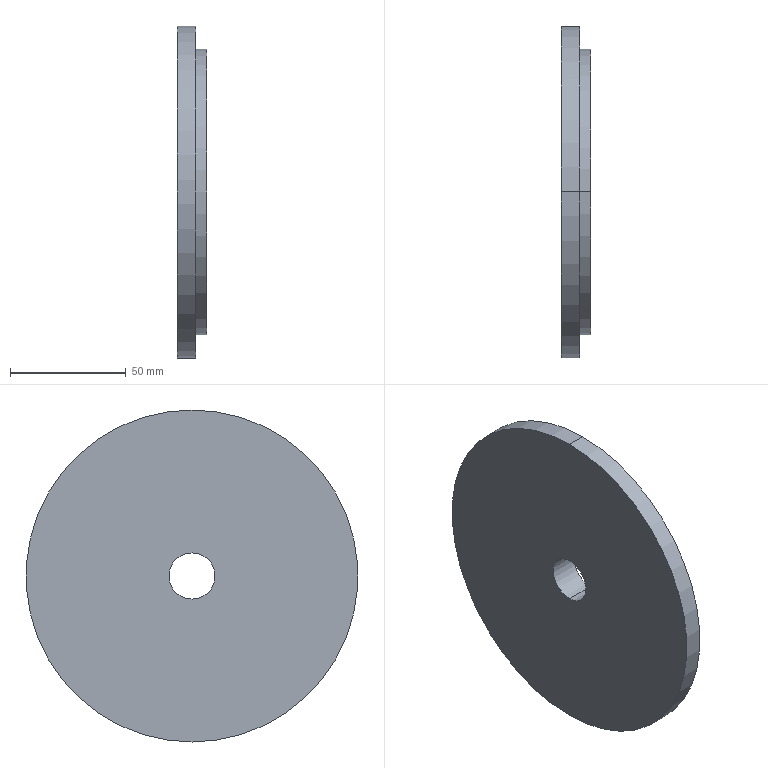Component | SolidWorks | MoldMountingPlate-1 | 1 solid | 9 faces | box 12.8 x 143.53 x 143.53 mm | volume 182945 mm3 | cylinder 6 | plane 3 | commonest cylinder face diameters 143.53 x2 123.53 x2 20 x2
build123d program:
from build123d import *


with BuildPart() as part:
    # Sketch1 → Revolve1 (revolve)
    with BuildSketch(Plane.XY, mode=Mode.PRIVATE) as revolve1_sk:
        Polygon((0, 10), (12.8, 10), (12.8, 61.765), (8, 61.765), (8, 71.765), (0, 71.765), align=None)
    revolve(revolve1_sk.sketch.rotate(Axis((0, 0, 0), (1, 0, 0)), 90), axis=Axis((0, 0, 0), (1, 0, 0)))


solid = part.part

# Placed as in the assembly
solid = solid.moved(Location((-6.743, 1299.706, 687.116), (0, 0, 0)))
STEP:
#1=COLOUR_RGB('',0.7922,0.8196,0.9333);
#2=FILL_AREA_STYLE_COLOUR('',#1);
#3=FILL_AREA_STYLE('',(#2));
#4=SURFACE_STYLE_FILL_AREA(#3);
#5=SURFACE_SIDE_STYLE('',(#4));
#6=SURFACE_STYLE_USAGE(.BOTH.,#5);
#7=PRESENTATION_STYLE_ASSIGNMENT((#6));
#8=CARTESIAN_POINT('',(0.04949,51.17,29.877));
#9=VERTEX_POINT('',#8);
#10=CARTESIAN_POINT('',(0.04949,51.17,24.226));
#11=VERTEX_POINT('',#10);
#12=CARTESIAN_POINT('',(0.04949,51.17,27.052));
#13=DIRECTION('',(-1.,0.,0.));
#14=DIRECTION('',(0.,0.,1.));
#15=AXIS2_PLACEMENT_3D('',#12,#13,#14);
#16=CIRCLE('',#15,2.825);
#17=EDGE_CURVE('',#9,#11,#16,.T.);
#18=ORIENTED_EDGE('',*,*,#17,.T.);
#19=CARTESIAN_POINT('',(-0.2655,51.17,24.226));
#20=VERTEX_POINT('',#19);
#21=CARTESIAN_POINT('',(-0.2655,51.17,24.226));
#22=DIRECTION('',(-1.,0.,0.));
#23=VECTOR('',#22,39.37);
#24=LINE('',#21,#23);
#25=EDGE_CURVE('',#11,#20,#24,.T.);
#26=ORIENTED_EDGE('',*,*,#25,.T.);
#27=CARTESIAN_POINT('',(-0.2655,51.17,29.877));
#28=VERTEX_POINT('',#27);
#29=CARTESIAN_POINT('',(-0.2655,51.17,27.052));
#30=DIRECTION('',(-1.,0.,0.));
#31=DIRECTION('',(0.,0.,1.));
#32=AXIS2_PLACEMENT_3D('',#29,#30,#31);
#33=CIRCLE('',#32,2.825);
#34=EDGE_CURVE('',#28,#20,#33,.T.);
#35=ORIENTED_EDGE('',*,*,#34,.F.);
#36=CARTESIAN_POINT('',(-0.2655,51.17,29.877));
#37=DIRECTION('',(-1.,0.,0.));
#38=VECTOR('',#37,39.37);
#39=LINE('',#36,#38);
#40=EDGE_CURVE('',#9,#28,#39,.T.);
#41=ORIENTED_EDGE('',*,*,#40,.F.);
#42=EDGE_LOOP('',(#18,#26,#35,#41));
#43=FACE_OUTER_BOUND('',#42,.T.);
#44=CARTESIAN_POINT('',(-0.2655,51.17,27.052));
#45=DIRECTION('',(-1.,0.,0.));
#46=DIRECTION('',(0.,0.,1.));
#47=AXIS2_PLACEMENT_3D('',#44,#45,#46);
#48=CYLINDRICAL_SURFACE('',#47,2.825);
#49=ADVANCED_FACE('',(#43),#48,.T.);
#50=CARTESIAN_POINT('',(0.2385,51.17,29.484));
#51=VERTEX_POINT('',#50);
#52=CARTESIAN_POINT('',(0.2385,51.17,24.62));
#53=VERTEX_POINT('',#52);
#54=CARTESIAN_POINT('',(0.2385,51.17,27.052));
#55=DIRECTION('',(-1.,0.,0.));
#56=DIRECTION('',(0.,0.,1.));
#57=AXIS2_PLACEMENT_3D('',#54,#55,#56);
#58=CIRCLE('',#57,2.432);
#59=EDGE_CURVE('',#51,#53,#58,.T.);
#60=ORIENTED_EDGE('',*,*,#59,.T.);
#61=CARTESIAN_POINT('',(0.04949,51.17,24.62));
#62=VERTEX_POINT('',#61);
#63=CARTESIAN_POINT('',(-0.2655,51.17,24.62));
#64=DIRECTION('',(-1.,0.,0.));
#65=VECTOR('',#64,39.37);
#66=LINE('',#63,#65);
#67=EDGE_CURVE('',#53,#62,#66,.T.);
#68=ORIENTED_EDGE('',*,*,#67,.T.);
#69=CARTESIAN_POINT('',(0.04949,51.17,29.484));
#70=VERTEX_POINT('',#69);
#71=CARTESIAN_POINT('',(0.04949,51.17,27.052));
#72=DIRECTION('',(-1.,0.,0.));
#73=DIRECTION('',(0.,0.,1.));
#74=AXIS2_PLACEMENT_3D('',#71,#72,#73);
#75=CIRCLE('',#74,2.432);
#76=EDGE_CURVE('',#70,#62,#75,.T.);
#77=ORIENTED_EDGE('',*,*,#76,.F.);
#78=CARTESIAN_POINT('',(-0.2655,51.17,29.484));
#79=DIRECTION('',(-1.,0.,0.));
#80=VECTOR('',#79,39.37);
#81=LINE('',#78,#80);
#82=EDGE_CURVE('',#51,#70,#81,.T.);
#83=ORIENTED_EDGE('',*,*,#82,.F.);
#84=EDGE_LOOP('',(#60,#68,#77,#83));
#85=FACE_OUTER_BOUND('',#84,.T.);
#86=CARTESIAN_POINT('',(-0.2655,51.17,27.052));
#87=DIRECTION('',(-1.,0.,0.));
#88=DIRECTION('',(0.,0.,1.));
#89=AXIS2_PLACEMENT_3D('',#86,#87,#88);
#90=CYLINDRICAL_SURFACE('',#89,2.432);
#91=ADVANCED_FACE('',(#85),#90,.T.);
#92=CARTESIAN_POINT('',(0.2385,51.17,26.658));
#93=VERTEX_POINT('',#92);
#94=CARTESIAN_POINT('',(0.2385,51.17,27.446));
#95=VERTEX_POINT('',#94);
#96=CARTESIAN_POINT('',(0.2385,51.17,27.052));
#97=DIRECTION('',(-1.,0.,0.));
#98=DIRECTION('',(0.,0.,1.));
#99=AXIS2_PLACEMENT_3D('',#96,#97,#98);
#100=CIRCLE('',#99,0.3937);
#101=EDGE_CURVE('',#93,#95,#100,.T.);
#102=ORIENTED_EDGE('',*,*,#101,.F.);
#103=CARTESIAN_POINT('',(-0.2655,51.17,26.658));
#104=VERTEX_POINT('',#103);
#105=CARTESIAN_POINT('',(-0.2655,51.17,26.658));
#106=DIRECTION('',(-1.,0.,0.));
#107=VECTOR('',#106,39.37);
#108=LINE('',#105,#107);
#109=EDGE_CURVE('',#93,#104,#108,.T.);
#110=ORIENTED_EDGE('',*,*,#109,.T.);
#111=CARTESIAN_POINT('',(-0.2655,51.17,27.446));
#112=VERTEX_POINT('',#111);
#113=CARTESIAN_POINT('',(-0.2655,51.17,27.052));
#114=DIRECTION('',(-1.,0.,0.));
#115=DIRECTION('',(0.,0.,1.));
#116=AXIS2_PLACEMENT_3D('',#113,#114,#115);
#117=CIRCLE('',#116,0.3937);
#118=EDGE_CURVE('',#104,#112,#117,.T.);
#119=ORIENTED_EDGE('',*,*,#118,.T.);
#120=CARTESIAN_POINT('',(-0.2655,51.17,27.446));
#121=DIRECTION('',(-1.,0.,0.));
#122=VECTOR('',#121,39.37);
#123=LINE('',#120,#122);
#124=EDGE_CURVE('',#95,#112,#123,.T.);
#125=ORIENTED_EDGE('',*,*,#124,.F.);
#126=EDGE_LOOP('',(#102,#110,#119,#125));
#127=FACE_OUTER_BOUND('',#126,.T.);
#128=CARTESIAN_POINT('',(-0.2655,51.17,27.052));
#129=DIRECTION('',(-1.,0.,0.));
#130=DIRECTION('',(0.,0.,1.));
#131=AXIS2_PLACEMENT_3D('',#128,#129,#130);
#132=CYLINDRICAL_SURFACE('',#131,0.3937);
#133=ADVANCED_FACE('',(#127),#132,.F.);
#134=CARTESIAN_POINT('',(-0.2655,51.17,27.052));
#135=DIRECTION('',(-1.,0.,0.));
#136=DIRECTION('',(0.,0.,1.));
#137=AXIS2_PLACEMENT_3D('',#134,#135,#136);
#138=CIRCLE('',#137,0.3937);
#139=EDGE_CURVE('',#112,#104,#138,.T.);
#140=ORIENTED_EDGE('',*,*,#139,.F.);
#141=ORIENTED_EDGE('',*,*,#118,.F.);
#142=EDGE_LOOP('',(#140,#141));
#143=FACE_BOUND('',#142,.T.);
#144=ORIENTED_EDGE('',*,*,#34,.T.);
#145=CARTESIAN_POINT('',(-0.2655,51.17,27.052));
#146=DIRECTION('',(-1.,0.,0.));
#147=DIRECTION('',(0.,0.,1.));
#148=AXIS2_PLACEMENT_3D('',#145,#146,#147);
#149=CIRCLE('',#148,2.825);
#150=EDGE_CURVE('',#20,#28,#149,.T.);
#151=ORIENTED_EDGE('',*,*,#150,.T.);
#152=EDGE_LOOP('',(#144,#151));
#153=FACE_OUTER_BOUND('',#152,.T.);
#154=CARTESIAN_POINT('',(-0.2655,53.995,27.052));
#155=DIRECTION('',(1.,0.,0.));
#156=DIRECTION('',(0.,0.,-1.));
#157=AXIS2_PLACEMENT_3D('',#154,#155,#156);
#158=PLANE('',#157);
#159=ADVANCED_FACE('',(#143,#153),#158,.F.);
#160=ORIENTED_EDGE('',*,*,#109,.F.);
#161=CARTESIAN_POINT('',(0.2385,51.17,27.052));
#162=DIRECTION('',(-1.,0.,0.));
#163=DIRECTION('',(0.,0.,1.));
#164=AXIS2_PLACEMENT_3D('',#161,#162,#163);
#165=CIRCLE('',#164,0.3937);
#166=EDGE_CURVE('',#95,#93,#165,.T.);
#167=ORIENTED_EDGE('',*,*,#166,.F.);
#168=ORIENTED_EDGE('',*,*,#124,.T.);
#169=ORIENTED_EDGE('',*,*,#139,.T.);
#170=EDGE_LOOP('',(#160,#167,#168,#169));
#171=FACE_OUTER_BOUND('',#170,.T.);
#172=CARTESIAN_POINT('',(-0.2655,51.17,27.052));
#173=DIRECTION('',(-1.,0.,0.));
#174=DIRECTION('',(0.,0.,1.));
#175=AXIS2_PLACEMENT_3D('',#172,#173,#174);
#176=CYLINDRICAL_SURFACE('',#175,0.3937);
#177=ADVANCED_FACE('',(#171),#176,.F.);
#178=ORIENTED_EDGE('',*,*,#59,.F.);
#179=CARTESIAN_POINT('',(0.2385,51.17,27.052));
#180=DIRECTION('',(-1.,0.,0.));
#181=DIRECTION('',(0.,0.,1.));
#182=AXIS2_PLACEMENT_3D('',#179,#180,#181);
#183=CIRCLE('',#182,2.432);
#184=EDGE_CURVE('',#53,#51,#183,.T.);
#185=ORIENTED_EDGE('',*,*,#184,.F.);
#186=EDGE_LOOP('',(#178,#185));
#187=FACE_OUTER_BOUND('',#186,.T.);
#188=ORIENTED_EDGE('',*,*,#166,.T.);
#189=ORIENTED_EDGE('',*,*,#101,.T.);
#190=EDGE_LOOP('',(#188,#189));
#191=FACE_BOUND('',#190,.T.);
#192=CARTESIAN_POINT('',(0.2385,51.563,27.052));
#193=DIRECTION('',(-1.,0.,0.));
#194=DIRECTION('',(0.,0.,1.));
#195=AXIS2_PLACEMENT_3D('',#192,#193,#194);
#196=PLANE('',#195);
#197=ADVANCED_FACE('',(#187,#191),#196,.F.);
#198=ORIENTED_EDGE('',*,*,#67,.F.);
#199=ORIENTED_EDGE('',*,*,#184,.T.);
#200=ORIENTED_EDGE('',*,*,#82,.T.);
#201=CARTESIAN_POINT('',(0.04949,51.17,27.052));
#202=DIRECTION('',(-1.,0.,0.));
#203=DIRECTION('',(0.,0.,1.));
#204=AXIS2_PLACEMENT_3D('',#201,#202,#203);
#205=CIRCLE('',#204,2.432);
#206=EDGE_CURVE('',#62,#70,#205,.T.);
#207=ORIENTED_EDGE('',*,*,#206,.F.);
#208=EDGE_LOOP('',(#198,#199,#200,#207));
#209=FACE_OUTER_BOUND('',#208,.T.);
#210=CARTESIAN_POINT('',(-0.2655,51.17,27.052));
#211=DIRECTION('',(-1.,0.,0.));
#212=DIRECTION('',(0.,0.,1.));
#213=AXIS2_PLACEMENT_3D('',#210,#211,#212);
#214=CYLINDRICAL_SURFACE('',#213,2.432);
#215=ADVANCED_FACE('',(#209),#214,.T.);
#216=ORIENTED_EDGE('',*,*,#17,.F.);
#217=CARTESIAN_POINT('',(0.04949,51.17,27.052));
#218=DIRECTION('',(-1.,0.,0.));
#219=DIRECTION('',(0.,0.,1.));
#220=AXIS2_PLACEMENT_3D('',#217,#218,#219);
#221=CIRCLE('',#220,2.825);
#222=EDGE_CURVE('',#11,#9,#221,.T.);
#223=ORIENTED_EDGE('',*,*,#222,.F.);
#224=EDGE_LOOP('',(#216,#223));
#225=FACE_OUTER_BOUND('',#224,.T.);
#226=ORIENTED_EDGE('',*,*,#76,.T.);
#227=ORIENTED_EDGE('',*,*,#206,.T.);
#228=EDGE_LOOP('',(#226,#227));
#229=FACE_BOUND('',#228,.T.);
#230=CARTESIAN_POINT('',(0.04949,53.601,27.052));
#231=DIRECTION('',(-1.,0.,0.));
#232=DIRECTION('',(0.,0.,1.));
#233=AXIS2_PLACEMENT_3D('',#230,#231,#232);
#234=PLANE('',#233);
#235=ADVANCED_FACE('',(#225,#229),#234,.F.);
#236=ORIENTED_EDGE('',*,*,#25,.F.);
#237=ORIENTED_EDGE('',*,*,#222,.T.);
#238=ORIENTED_EDGE('',*,*,#40,.T.);
#239=ORIENTED_EDGE('',*,*,#150,.F.);
#240=EDGE_LOOP('',(#236,#237,#238,#239));
#241=FACE_OUTER_BOUND('',#240,.T.);
#242=CARTESIAN_POINT('',(-0.2655,51.17,27.052));
#243=DIRECTION('',(-1.,0.,0.));
#244=DIRECTION('',(0.,0.,1.));
#245=AXIS2_PLACEMENT_3D('',#242,#243,#244);
#246=CYLINDRICAL_SURFACE('',#245,2.825);
#247=ADVANCED_FACE('',(#241),#246,.T.);
#248=CLOSED_SHELL('',(#49,#91,#133,#159,#177,#197,#215,#235,#247));
#249=MANIFOLD_SOLID_BREP('',#248);
#250=STYLED_ITEM('',(#7),#249);
#251=(LENGTH_UNIT()NAMED_UNIT(*)SI_UNIT($,.METRE.));
#252=LENGTH_MEASURE_WITH_UNIT(LENGTH_MEASURE(0.0254),#251);
#253=DIMENSIONAL_EXPONENTS(1.,0.,0.,0.,0.,0.,0.);
#254=(CONVERSION_BASED_UNIT('',#252)LENGTH_UNIT()NAMED_UNIT(#253));
#255=UNCERTAINTY_MEASURE_WITH_UNIT(LENGTH_MEASURE(0.00001),#254,'','');
#256=(NAMED_UNIT(*)PLANE_ANGLE_UNIT()SI_UNIT($,.RADIAN.));
#257=(NAMED_UNIT(*)SI_UNIT($,.STERADIAN.)SOLID_ANGLE_UNIT());
#258=(GEOMETRIC_REPRESENTATION_CONTEXT(3)GLOBAL_UNCERTAINTY_ASSIGNED_CONTEXT((#255))GLOBAL_UNIT_ASSIGNED_CONTEXT((#254,#256,#257))REPRESENTATION_CONTEXT('',''));
#259=MECHANICAL_DESIGN_GEOMETRIC_PRESENTATION_REPRESENTATION('',(#250),#258);
#260=PRESENTATION_LAYER_ASSIGNMENT('','',(#250));
#261=CARTESIAN_POINT('',(0.,0.,0.));
#262=DIRECTION('',(0.,0.,1.));
#263=DIRECTION('',(1.,0.,0.));
#264=AXIS2_PLACEMENT_3D('',#261,#262,#263);
#265=(LENGTH_UNIT()NAMED_UNIT(*)SI_UNIT($,.METRE.));
#266=LENGTH_MEASURE_WITH_UNIT(LENGTH_MEASURE(0.0254),#265);
#267=DIMENSIONAL_EXPONENTS(1.,0.,0.,0.,0.,0.,0.);
#268=(CONVERSION_BASED_UNIT('',#266)LENGTH_UNIT()NAMED_UNIT(#267));
#269=UNCERTAINTY_MEASURE_WITH_UNIT(LENGTH_MEASURE(0.00001),#268,'','');
#270=(NAMED_UNIT(*)PLANE_ANGLE_UNIT()SI_UNIT($,.RADIAN.));
#271=(NAMED_UNIT(*)SI_UNIT($,.STERADIAN.)SOLID_ANGLE_UNIT());
#272=(GEOMETRIC_REPRESENTATION_CONTEXT(3)GLOBAL_UNCERTAINTY_ASSIGNED_CONTEXT((#269))GLOBAL_UNIT_ASSIGNED_CONTEXT((#268,#270,#271))REPRESENTATION_CONTEXT('',''));
#273=ADVANCED_BREP_SHAPE_REPRESENTATION('',(#249,#264),#272);